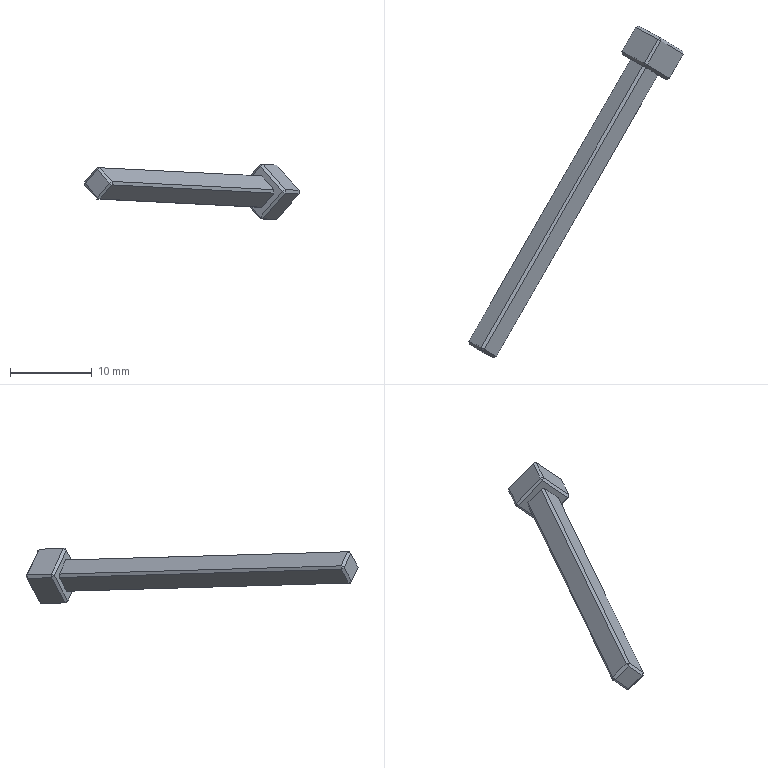Component | SolidWorks | 6z0-123-1 | 1 solid | 46 faces | box 26.14 x 40.54 x 6.74 mm | volume 422 mm3 | plane 44 | cylinder 2 | commonest cylinder face diameters 4.2 x2
STEP:
#1=COLOUR_RGB('',0.7922,0.8196,0.9333);
#2=FILL_AREA_STYLE_COLOUR('',#1);
#3=FILL_AREA_STYLE('',(#2));
#4=SURFACE_STYLE_FILL_AREA(#3);
#5=SURFACE_SIDE_STYLE('',(#4));
#6=SURFACE_STYLE_USAGE(.BOTH.,#5);
#7=PRESENTATION_STYLE_ASSIGNMENT((#6));
#8=CARTESIAN_POINT('',(-3.495,-3.817,3.283));
#9=VERTEX_POINT('',#8);
#10=CARTESIAN_POINT('',(-3.394,-3.878,3.168));
#11=VERTEX_POINT('',#10);
#12=CARTESIAN_POINT('',(-3.445,-3.847,3.225));
#13=DIRECTION('',(0.4977,0.867,-0.02519));
#14=DIRECTION('',(0.6119,-0.3716,-0.6982));
#15=AXIS2_PLACEMENT_3D('',#12,#13,#14);
#16=CIRCLE('',#15,0.08268);
#17=EDGE_CURVE('',#9,#11,#16,.T.);
#18=ORIENTED_EDGE('',*,*,#17,.F.);
#19=CARTESIAN_POINT('',(-3.456,-3.748,3.281));
#20=VERTEX_POINT('',#19);
#21=CARTESIAN_POINT('',(-3.495,-3.817,3.283));
#22=DIRECTION('',(0.4977,0.867,-0.02519));
#23=VECTOR('',#22,39.37);
#24=LINE('',#21,#23);
#25=EDGE_CURVE('',#9,#20,#24,.T.);
#26=ORIENTED_EDGE('',*,*,#25,.T.);
#27=CARTESIAN_POINT('',(-3.355,-3.81,3.166));
#28=VERTEX_POINT('',#27);
#29=CARTESIAN_POINT('',(-3.406,-3.779,3.223));
#30=DIRECTION('',(0.4977,0.867,-0.02519));
#31=DIRECTION('',(0.6119,-0.3716,-0.6982));
#32=AXIS2_PLACEMENT_3D('',#29,#30,#31);
#33=CIRCLE('',#32,0.08268);
#34=EDGE_CURVE('',#20,#28,#33,.T.);
#35=ORIENTED_EDGE('',*,*,#34,.T.);
#36=CARTESIAN_POINT('',(-3.394,-3.878,3.168));
#37=DIRECTION('',(0.4977,0.867,-0.02519));
#38=VECTOR('',#37,39.37);
#39=LINE('',#36,#38);
#40=EDGE_CURVE('',#11,#28,#39,.T.);
#41=ORIENTED_EDGE('',*,*,#40,.F.);
#42=EDGE_LOOP('',(#18,#26,#35,#41));
#43=FACE_OUTER_BOUND('',#42,.T.);
#44=CARTESIAN_POINT('',(-3.445,-3.847,3.225));
#45=DIRECTION('',(0.4977,0.867,-0.02519));
#46=DIRECTION('',(0.6119,-0.3716,-0.6982));
#47=AXIS2_PLACEMENT_3D('',#44,#45,#46);
#48=CYLINDRICAL_SURFACE('',#47,0.08268);
#49=ADVANCED_FACE('',(#43),#48,.F.);
#50=CARTESIAN_POINT('',(-3.484,-3.919,3.105));
#51=VERTEX_POINT('',#50);
#52=CARTESIAN_POINT('',(-3.378,-3.977,3.229));
#53=VERTEX_POINT('',#52);
#54=CARTESIAN_POINT('',(-3.371,-3.981,3.237));
#55=DIRECTION('',(0.6147,-0.3321,0.7154));
#56=VECTOR('',#55,39.37);
#57=LINE('',#54,#56);
#58=EDGE_CURVE('',#51,#53,#57,.T.);
#59=ORIENTED_EDGE('',*,*,#58,.T.);
#60=CARTESIAN_POINT('',(-3.484,-3.912,3.35));
#61=VERTEX_POINT('',#60);
#62=CARTESIAN_POINT('',(-3.491,-3.908,3.358));
#63=DIRECTION('',(-0.6119,0.3716,0.6982));
#64=VECTOR('',#63,39.37);
#65=LINE('',#62,#64);
#66=EDGE_CURVE('',#53,#61,#65,.T.);
#67=ORIENTED_EDGE('',*,*,#66,.T.);
#68=CARTESIAN_POINT('',(-3.59,-3.855,3.226));
#69=VERTEX_POINT('',#68);
#70=CARTESIAN_POINT('',(-3.598,-3.851,3.217));
#71=DIRECTION('',(-0.6147,0.3321,-0.7154));
#72=VECTOR('',#71,39.37);
#73=LINE('',#70,#72);
#74=EDGE_CURVE('',#61,#69,#73,.T.);
#75=ORIENTED_EDGE('',*,*,#74,.T.);
#76=CARTESIAN_POINT('',(-3.477,-3.924,3.097));
#77=DIRECTION('',(0.6119,-0.3716,-0.6982));
#78=VECTOR('',#77,39.37);
#79=LINE('',#76,#78);
#80=EDGE_CURVE('',#69,#51,#79,.T.);
#81=ORIENTED_EDGE('',*,*,#80,.T.);
#82=EDGE_LOOP('',(#59,#67,#75,#81));
#83=FACE_OUTER_BOUND('',#82,.T.);
#84=CARTESIAN_POINT('',(-3.549,-3.879,3.218));
#85=VERTEX_POINT('',#84);
#86=CARTESIAN_POINT('',(-3.491,-3.914,3.152));
#87=VERTEX_POINT('',#86);
#88=CARTESIAN_POINT('',(-3.484,-3.918,3.144));
#89=DIRECTION('',(0.6119,-0.3716,-0.6982));
#90=VECTOR('',#89,39.37);
#91=LINE('',#88,#90);
#92=EDGE_CURVE('',#85,#87,#91,.T.);
#93=ORIENTED_EDGE('',*,*,#92,.F.);
#94=CARTESIAN_POINT('',(-3.549,-3.878,3.235));
#95=VERTEX_POINT('',#94);
#96=CARTESIAN_POINT('',(-3.549,-3.879,3.218));
#97=DIRECTION('',(0.001966,0.02792,0.9996));
#98=VECTOR('',#97,39.37);
#99=LINE('',#96,#98);
#100=EDGE_CURVE('',#85,#95,#99,.T.);
#101=ORIENTED_EDGE('',*,*,#100,.T.);
#102=CARTESIAN_POINT('',(-3.491,-3.909,3.302));
#103=VERTEX_POINT('',#102);
#104=CARTESIAN_POINT('',(-3.556,-3.874,3.226));
#105=DIRECTION('',(-0.6147,0.3321,-0.7154));
#106=VECTOR('',#105,39.37);
#107=LINE('',#104,#106);
#108=EDGE_CURVE('',#103,#95,#107,.T.);
#109=ORIENTED_EDGE('',*,*,#108,.F.);
#110=CARTESIAN_POINT('',(-3.477,-3.918,3.302));
#111=VERTEX_POINT('',#110);
#112=CARTESIAN_POINT('',(-3.491,-3.909,3.302));
#113=DIRECTION('',(0.8673,-0.4976,0.01219));
#114=VECTOR('',#113,39.37);
#115=LINE('',#112,#114);
#116=EDGE_CURVE('',#103,#111,#115,.T.);
#117=ORIENTED_EDGE('',*,*,#116,.T.);
#118=CARTESIAN_POINT('',(-3.419,-3.953,3.237));
#119=VERTEX_POINT('',#118);
#120=CARTESIAN_POINT('',(-3.412,-3.957,3.228));
#121=DIRECTION('',(-0.6119,0.3716,0.6982));
#122=VECTOR('',#121,39.37);
#123=LINE('',#120,#122);
#124=EDGE_CURVE('',#119,#111,#123,.T.);
#125=ORIENTED_EDGE('',*,*,#124,.F.);
#126=CARTESIAN_POINT('',(-3.419,-3.953,3.22));
#127=VERTEX_POINT('',#126);
#128=CARTESIAN_POINT('',(-3.419,-3.953,3.237));
#129=DIRECTION('',(-0.001966,-0.02792,-0.9996));
#130=VECTOR('',#129,39.37);
#131=LINE('',#128,#130);
#132=EDGE_CURVE('',#119,#127,#131,.T.);
#133=ORIENTED_EDGE('',*,*,#132,.T.);
#134=CARTESIAN_POINT('',(-3.477,-3.922,3.152));
#135=VERTEX_POINT('',#134);
#136=CARTESIAN_POINT('',(-3.484,-3.918,3.144));
#137=DIRECTION('',(0.6147,-0.3321,0.7154));
#138=VECTOR('',#137,39.37);
#139=LINE('',#136,#138);
#140=EDGE_CURVE('',#135,#127,#139,.T.);
#141=ORIENTED_EDGE('',*,*,#140,.F.);
#142=CARTESIAN_POINT('',(-3.477,-3.922,3.152));
#143=DIRECTION('',(-0.8673,0.4976,-0.01219));
#144=VECTOR('',#143,39.37);
#145=LINE('',#142,#144);
#146=EDGE_CURVE('',#135,#87,#145,.T.);
#147=ORIENTED_EDGE('',*,*,#146,.T.);
#148=EDGE_LOOP('',(#93,#101,#109,#117,#125,#133,#141,#147));
#149=FACE_BOUND('',#148,.T.);
#150=CARTESIAN_POINT('',(-3.484,-3.916,3.227));
#151=DIRECTION('',(-0.4977,-0.867,0.02519));
#152=DIRECTION('',(-0.6119,0.3716,0.6982));
#153=AXIS2_PLACEMENT_3D('',#150,#151,#152);
#154=PLANE('',#153);
#155=ADVANCED_FACE('',(#83,#149),#154,.T.);
#156=CARTESIAN_POINT('',(-3.525,-3.724,3.23));
#157=VERTEX_POINT('',#156);
#158=CARTESIAN_POINT('',(-3.592,-3.84,3.234));
#159=VERTEX_POINT('',#158);
#160=CARTESIAN_POINT('',(-3.598,-3.85,3.234));
#161=DIRECTION('',(-0.4977,-0.867,0.02519));
#162=VECTOR('',#161,39.37);
#163=LINE('',#160,#162);
#164=EDGE_CURVE('',#157,#159,#163,.T.);
#165=ORIENTED_EDGE('',*,*,#164,.T.);
#166=CARTESIAN_POINT('',(-3.485,-3.898,3.358));
#167=VERTEX_POINT('',#166);
#168=CARTESIAN_POINT('',(-3.478,-3.902,3.366));
#169=DIRECTION('',(0.6147,-0.3321,0.7154));
#170=VECTOR('',#169,39.37);
#171=LINE('',#168,#170);
#172=EDGE_CURVE('',#159,#167,#171,.T.);
#173=ORIENTED_EDGE('',*,*,#172,.T.);
#174=CARTESIAN_POINT('',(-3.419,-3.782,3.354));
#175=VERTEX_POINT('',#174);
#176=CARTESIAN_POINT('',(-3.491,-3.908,3.358));
#177=DIRECTION('',(0.4977,0.867,-0.02519));
#178=VECTOR('',#177,39.37);
#179=LINE('',#176,#178);
#180=EDGE_CURVE('',#167,#175,#179,.T.);
#181=ORIENTED_EDGE('',*,*,#180,.T.);
#182=CARTESIAN_POINT('',(-3.532,-3.72,3.222));
#183=DIRECTION('',(-0.6147,0.3321,-0.7154));
#184=VECTOR('',#183,39.37);
#185=LINE('',#182,#184);
#186=EDGE_CURVE('',#175,#157,#185,.T.);
#187=ORIENTED_EDGE('',*,*,#186,.T.);
#188=EDGE_LOOP('',(#165,#173,#181,#187));
#189=FACE_OUTER_BOUND('',#188,.T.);
#190=CARTESIAN_POINT('',(-3.605,-3.846,3.226));
#191=DIRECTION('',(0.6119,-0.3716,-0.6982));
#192=DIRECTION('',(0.6147,-0.3321,0.7154));
#193=AXIS2_PLACEMENT_3D('',#190,#191,#192);
#194=PLANE('',#193);
#195=ADVANCED_FACE('',(#189),#194,.F.);
#196=CARTESIAN_POINT('',(-3.486,-3.905,3.096));
#197=VERTEX_POINT('',#196);
#198=CARTESIAN_POINT('',(-3.592,-3.841,3.217));
#199=VERTEX_POINT('',#198);
#200=CARTESIAN_POINT('',(-3.599,-3.836,3.225));
#201=DIRECTION('',(-0.6119,0.3716,0.6982));
#202=VECTOR('',#201,39.37);
#203=LINE('',#200,#202);
#204=EDGE_CURVE('',#197,#199,#203,.T.);
#205=ORIENTED_EDGE('',*,*,#204,.T.);
#206=CARTESIAN_POINT('',(-3.525,-3.725,3.214));
#207=VERTEX_POINT('',#206);
#208=CARTESIAN_POINT('',(-3.598,-3.851,3.217));
#209=DIRECTION('',(0.4977,0.867,-0.02519));
#210=VECTOR('',#209,39.37);
#211=LINE('',#208,#210);
#212=EDGE_CURVE('',#199,#207,#211,.T.);
#213=ORIENTED_EDGE('',*,*,#212,.T.);
#214=CARTESIAN_POINT('',(-3.419,-3.789,3.093));
#215=VERTEX_POINT('',#214);
#216=CARTESIAN_POINT('',(-3.412,-3.793,3.084));
#217=DIRECTION('',(0.6119,-0.3716,-0.6982));
#218=VECTOR('',#217,39.37);
#219=LINE('',#216,#218);
#220=EDGE_CURVE('',#207,#215,#219,.T.);
#221=ORIENTED_EDGE('',*,*,#220,.T.);
#222=CARTESIAN_POINT('',(-3.492,-3.915,3.096));
#223=DIRECTION('',(-0.4977,-0.867,0.02519));
#224=VECTOR('',#223,39.37);
#225=LINE('',#222,#224);
#226=EDGE_CURVE('',#215,#197,#225,.T.);
#227=ORIENTED_EDGE('',*,*,#226,.T.);
#228=EDGE_LOOP('',(#205,#213,#221,#227));
#229=FACE_OUTER_BOUND('',#228,.T.);
#230=CARTESIAN_POINT('',(-3.484,-3.92,3.088));
#231=DIRECTION('',(0.6147,-0.3321,0.7154));
#232=DIRECTION('',(0.4977,0.867,-0.02519));
#233=AXIS2_PLACEMENT_3D('',#230,#231,#232);
#234=PLANE('',#233);
#235=ADVANCED_FACE('',(#229),#234,.F.);
#236=CARTESIAN_POINT('',(-3.405,-3.797,3.093));
#237=VERTEX_POINT('',#236);
#238=CARTESIAN_POINT('',(-3.298,-3.855,3.217));
#239=VERTEX_POINT('',#238);
#240=CARTESIAN_POINT('',(-3.412,-3.793,3.084));
#241=DIRECTION('',(0.6147,-0.3321,0.7154));
#242=VECTOR('',#241,39.37);
#243=LINE('',#240,#242);
#244=EDGE_CURVE('',#237,#239,#243,.T.);
#245=ORIENTED_EDGE('',*,*,#244,.T.);
#246=CARTESIAN_POINT('',(-3.365,-3.971,3.22));
#247=VERTEX_POINT('',#246);
#248=CARTESIAN_POINT('',(-3.371,-3.981,3.22));
#249=DIRECTION('',(-0.4977,-0.867,0.02519));
#250=VECTOR('',#249,39.37);
#251=LINE('',#248,#250);
#252=EDGE_CURVE('',#239,#247,#251,.T.);
#253=ORIENTED_EDGE('',*,*,#252,.T.);
#254=CARTESIAN_POINT('',(-3.471,-3.913,3.096));
#255=VERTEX_POINT('',#254);
#256=CARTESIAN_POINT('',(-3.478,-3.909,3.088));
#257=DIRECTION('',(-0.6147,0.3321,-0.7154));
#258=VECTOR('',#257,39.37);
#259=LINE('',#256,#258);
#260=EDGE_CURVE('',#247,#255,#259,.T.);
#261=ORIENTED_EDGE('',*,*,#260,.T.);
#262=CARTESIAN_POINT('',(-3.477,-3.924,3.097));
#263=DIRECTION('',(0.4977,0.867,-0.02519));
#264=VECTOR('',#263,39.37);
#265=LINE('',#262,#264);
#266=EDGE_CURVE('',#255,#237,#265,.T.);
#267=ORIENTED_EDGE('',*,*,#266,.T.);
#268=EDGE_LOOP('',(#245,#253,#261,#267));
#269=FACE_OUTER_BOUND('',#268,.T.);
#270=CARTESIAN_POINT('',(-3.484,-3.92,3.088));
#271=DIRECTION('',(-0.6119,0.3716,0.6982));
#272=DIRECTION('',(-0.6147,0.3321,-0.7154));
#273=AXIS2_PLACEMENT_3D('',#270,#271,#272);
#274=PLANE('',#273);
#275=ADVANCED_FACE('',(#269),#274,.F.);
#276=CARTESIAN_POINT('',(-3.471,-3.906,3.358));
#277=VERTEX_POINT('',#276);
#278=CARTESIAN_POINT('',(-3.365,-3.97,3.237));
#279=VERTEX_POINT('',#278);
#280=CARTESIAN_POINT('',(-3.357,-3.975,3.229));
#281=DIRECTION('',(0.6119,-0.3716,-0.6982));
#282=VECTOR('',#281,39.37);
#283=LINE('',#280,#282);
#284=EDGE_CURVE('',#277,#279,#283,.T.);
#285=ORIENTED_EDGE('',*,*,#284,.T.);
#286=CARTESIAN_POINT('',(-3.298,-3.854,3.234));
#287=VERTEX_POINT('',#286);
#288=CARTESIAN_POINT('',(-3.371,-3.981,3.237));
#289=DIRECTION('',(0.4977,0.867,-0.02519));
#290=VECTOR('',#289,39.37);
#291=LINE('',#288,#290);
#292=EDGE_CURVE('',#279,#287,#291,.T.);
#293=ORIENTED_EDGE('',*,*,#292,.T.);
#294=CARTESIAN_POINT('',(-3.404,-3.79,3.354));
#295=VERTEX_POINT('',#294);
#296=CARTESIAN_POINT('',(-3.291,-3.859,3.225));
#297=DIRECTION('',(-0.6119,0.3716,0.6982));
#298=VECTOR('',#297,39.37);
#299=LINE('',#296,#298);
#300=EDGE_CURVE('',#287,#295,#299,.T.);
#301=ORIENTED_EDGE('',*,*,#300,.T.);
#302=CARTESIAN_POINT('',(-3.477,-3.916,3.358));
#303=DIRECTION('',(-0.4977,-0.867,0.02519));
#304=VECTOR('',#303,39.37);
#305=LINE('',#302,#304);
#306=EDGE_CURVE('',#295,#277,#305,.T.);
#307=ORIENTED_EDGE('',*,*,#306,.T.);
#308=EDGE_LOOP('',(#285,#293,#301,#307));
#309=FACE_OUTER_BOUND('',#308,.T.);
#310=CARTESIAN_POINT('',(-3.363,-3.985,3.229));
#311=DIRECTION('',(-0.6147,0.3321,-0.7154));
#312=DIRECTION('',(-0.4977,-0.867,0.02519));
#313=AXIS2_PLACEMENT_3D('',#310,#311,#312);
#314=PLANE('',#313);
#315=ADVANCED_FACE('',(#309),#314,.F.);
#316=CARTESIAN_POINT('',(-3.512,-3.718,3.222));
#317=VERTEX_POINT('',#316);
#318=CARTESIAN_POINT('',(-3.405,-3.776,3.346));
#319=VERTEX_POINT('',#318);
#320=CARTESIAN_POINT('',(-3.459,-3.747,3.284));
#321=DIRECTION('',(0.6147,-0.3321,0.7154));
#322=VECTOR('',#321,39.37);
#323=LINE('',#320,#322);
#324=EDGE_CURVE('',#317,#319,#323,.T.);
#325=ORIENTED_EDGE('',*,*,#324,.T.);
#326=CARTESIAN_POINT('',(-3.299,-3.84,3.225));
#327=VERTEX_POINT('',#326);
#328=CARTESIAN_POINT('',(-3.352,-3.808,3.285));
#329=DIRECTION('',(0.6119,-0.3716,-0.6982));
#330=VECTOR('',#329,39.37);
#331=LINE('',#328,#330);
#332=EDGE_CURVE('',#319,#327,#331,.T.);
#333=ORIENTED_EDGE('',*,*,#332,.T.);
#334=CARTESIAN_POINT('',(-3.406,-3.783,3.101));
#335=VERTEX_POINT('',#334);
#336=CARTESIAN_POINT('',(-3.353,-3.811,3.163));
#337=DIRECTION('',(-0.6147,0.3321,-0.7154));
#338=VECTOR('',#337,39.37);
#339=LINE('',#336,#338);
#340=EDGE_CURVE('',#327,#335,#339,.T.);
#341=ORIENTED_EDGE('',*,*,#340,.T.);
#342=CARTESIAN_POINT('',(-3.459,-3.75,3.161));
#343=DIRECTION('',(-0.6119,0.3716,0.6982));
#344=VECTOR('',#343,39.37);
#345=LINE('',#342,#344);
#346=EDGE_CURVE('',#335,#317,#345,.T.);
#347=ORIENTED_EDGE('',*,*,#346,.T.);
#348=EDGE_LOOP('',(#325,#333,#341,#347));
#349=FACE_OUTER_BOUND('',#348,.T.);
#350=CARTESIAN_POINT('',(-3.406,-3.779,3.223));
#351=DIRECTION('',(0.4977,0.867,-0.02519));
#352=DIRECTION('',(0.6119,-0.3716,-0.6982));
#353=AXIS2_PLACEMENT_3D('',#350,#351,#352);
#354=CIRCLE('',#353,0.08268);
#355=EDGE_CURVE('',#28,#20,#354,.T.);
#356=ORIENTED_EDGE('',*,*,#355,.F.);
#357=ORIENTED_EDGE('',*,*,#34,.F.);
#358=EDGE_LOOP('',(#356,#357));
#359=FACE_BOUND('',#358,.T.);
#360=CARTESIAN_POINT('',(-3.406,-3.779,3.223));
#361=DIRECTION('',(-0.4977,-0.867,0.02519));
#362=DIRECTION('',(-0.6119,0.3716,0.6982));
#363=AXIS2_PLACEMENT_3D('',#360,#361,#362);
#364=PLANE('',#363);
#365=ADVANCED_FACE('',(#349,#359),#364,.F.);
#366=CARTESIAN_POINT('',(-4.327,-5.233,3.274));
#367=VERTEX_POINT('',#366);
#368=CARTESIAN_POINT('',(-4.269,-5.265,3.342));
#369=VERTEX_POINT('',#368);
#370=CARTESIAN_POINT('',(-4.262,-5.268,3.35));
#371=DIRECTION('',(0.6147,-0.3321,0.7154));
#372=VECTOR('',#371,39.37);
#373=LINE('',#370,#372);
#374=EDGE_CURVE('',#367,#369,#373,.T.);
#375=ORIENTED_EDGE('',*,*,#374,.T.);
#376=CARTESIAN_POINT('',(-4.275,-5.275,3.342));
#377=DIRECTION('',(0.4977,0.867,-0.02519));
#378=VECTOR('',#377,39.37);
#379=LINE('',#376,#378);
#380=EDGE_CURVE('',#369,#103,#379,.T.);
#381=ORIENTED_EDGE('',*,*,#380,.T.);
#382=ORIENTED_EDGE('',*,*,#108,.T.);
#383=CARTESIAN_POINT('',(-4.333,-5.243,3.274));
#384=DIRECTION('',(-0.4977,-0.867,0.02519));
#385=VECTOR('',#384,39.37);
#386=LINE('',#383,#385);
#387=EDGE_CURVE('',#95,#367,#386,.T.);
#388=ORIENTED_EDGE('',*,*,#387,.T.);
#389=EDGE_LOOP('',(#375,#381,#382,#388));
#390=FACE_OUTER_BOUND('',#389,.T.);
#391=CARTESIAN_POINT('',(-4.34,-5.239,3.266));
#392=DIRECTION('',(0.6119,-0.3716,-0.6982));
#393=DIRECTION('',(0.6147,-0.3321,0.7154));
#394=AXIS2_PLACEMENT_3D('',#391,#392,#393);
#395=PLANE('',#394);
#396=ADVANCED_FACE('',(#390),#395,.F.);
#397=ORIENTED_EDGE('',*,*,#92,.T.);
#398=CARTESIAN_POINT('',(-4.269,-5.269,3.191));
#399=VERTEX_POINT('',#398);
#400=CARTESIAN_POINT('',(-4.275,-5.279,3.192));
#401=DIRECTION('',(-0.4977,-0.867,0.02519));
#402=VECTOR('',#401,39.37);
#403=LINE('',#400,#402);
#404=EDGE_CURVE('',#87,#399,#403,.T.);
#405=ORIENTED_EDGE('',*,*,#404,.T.);
#406=CARTESIAN_POINT('',(-4.327,-5.234,3.257));
#407=VERTEX_POINT('',#406);
#408=CARTESIAN_POINT('',(-4.334,-5.229,3.266));
#409=DIRECTION('',(-0.6119,0.3716,0.6982));
#410=VECTOR('',#409,39.37);
#411=LINE('',#408,#410);
#412=EDGE_CURVE('',#399,#407,#411,.T.);
#413=ORIENTED_EDGE('',*,*,#412,.T.);
#414=CARTESIAN_POINT('',(-4.333,-5.244,3.258));
#415=DIRECTION('',(0.4977,0.867,-0.02519));
#416=VECTOR('',#415,39.37);
#417=LINE('',#414,#416);
#418=EDGE_CURVE('',#407,#85,#417,.T.);
#419=ORIENTED_EDGE('',*,*,#418,.T.);
#420=EDGE_LOOP('',(#397,#405,#413,#419));
#421=FACE_OUTER_BOUND('',#420,.T.);
#422=CARTESIAN_POINT('',(-4.268,-5.283,3.183));
#423=DIRECTION('',(0.6147,-0.3321,0.7154));
#424=DIRECTION('',(0.4977,0.867,-0.02519));
#425=AXIS2_PLACEMENT_3D('',#422,#423,#424);
#426=PLANE('',#425);
#427=ADVANCED_FACE('',(#421),#426,.F.);
#428=ORIENTED_EDGE('',*,*,#140,.T.);
#429=CARTESIAN_POINT('',(-4.197,-5.308,3.259));
#430=VERTEX_POINT('',#429);
#431=CARTESIAN_POINT('',(-4.203,-5.319,3.259));
#432=DIRECTION('',(-0.4977,-0.867,0.02519));
#433=VECTOR('',#432,39.37);
#434=LINE('',#431,#433);
#435=EDGE_CURVE('',#127,#430,#434,.T.);
#436=ORIENTED_EDGE('',*,*,#435,.T.);
#437=CARTESIAN_POINT('',(-4.255,-5.277,3.192));
#438=VERTEX_POINT('',#437);
#439=CARTESIAN_POINT('',(-4.262,-5.273,3.183));
#440=DIRECTION('',(-0.6147,0.3321,-0.7154));
#441=VECTOR('',#440,39.37);
#442=LINE('',#439,#441);
#443=EDGE_CURVE('',#430,#438,#442,.T.);
#444=ORIENTED_EDGE('',*,*,#443,.T.);
#445=CARTESIAN_POINT('',(-4.261,-5.287,3.192));
#446=DIRECTION('',(0.4977,0.867,-0.02519));
#447=VECTOR('',#446,39.37);
#448=LINE('',#445,#447);
#449=EDGE_CURVE('',#438,#135,#448,.T.);
#450=ORIENTED_EDGE('',*,*,#449,.T.);
#451=EDGE_LOOP('',(#428,#436,#444,#450));
#452=FACE_OUTER_BOUND('',#451,.T.);
#453=CARTESIAN_POINT('',(-4.268,-5.283,3.183));
#454=DIRECTION('',(-0.6119,0.3716,0.6982));
#455=DIRECTION('',(-0.6147,0.3321,-0.7154));
#456=AXIS2_PLACEMENT_3D('',#453,#454,#455);
#457=PLANE('',#456);
#458=ADVANCED_FACE('',(#452),#457,.F.);
#459=CARTESIAN_POINT('',(-4.255,-5.273,3.342));
#460=VERTEX_POINT('',#459);
#461=CARTESIAN_POINT('',(-4.197,-5.308,3.276));
#462=VERTEX_POINT('',#461);
#463=CARTESIAN_POINT('',(-4.19,-5.312,3.268));
#464=DIRECTION('',(0.6119,-0.3716,-0.6982));
#465=VECTOR('',#464,39.37);
#466=LINE('',#463,#465);
#467=EDGE_CURVE('',#460,#462,#466,.T.);
#468=ORIENTED_EDGE('',*,*,#467,.T.);
#469=CARTESIAN_POINT('',(-4.203,-5.318,3.276));
#470=DIRECTION('',(0.4977,0.867,-0.02519));
#471=VECTOR('',#470,39.37);
#472=LINE('',#469,#471);
#473=EDGE_CURVE('',#462,#119,#472,.T.);
#474=ORIENTED_EDGE('',*,*,#473,.T.);
#475=ORIENTED_EDGE('',*,*,#124,.T.);
#476=CARTESIAN_POINT('',(-4.26,-5.283,3.342));
#477=DIRECTION('',(-0.4977,-0.867,0.02519));
#478=VECTOR('',#477,39.37);
#479=LINE('',#476,#478);
#480=EDGE_CURVE('',#111,#460,#479,.T.);
#481=ORIENTED_EDGE('',*,*,#480,.T.);
#482=EDGE_LOOP('',(#468,#474,#475,#481));
#483=FACE_OUTER_BOUND('',#482,.T.);
#484=CARTESIAN_POINT('',(-4.195,-5.323,3.268));
#485=DIRECTION('',(-0.6147,0.3321,-0.7154));
#486=DIRECTION('',(-0.4977,-0.867,0.02519));
#487=AXIS2_PLACEMENT_3D('',#484,#485,#486);
#488=PLANE('',#487);
#489=ADVANCED_FACE('',(#483),#488,.F.);
#490=CARTESIAN_POINT('',(-4.268,-5.279,3.334));
#491=VERTEX_POINT('',#490);
#492=CARTESIAN_POINT('',(-4.326,-5.248,3.266));
#493=VERTEX_POINT('',#492);
#494=CARTESIAN_POINT('',(-4.333,-5.244,3.258));
#495=DIRECTION('',(-0.6147,0.3321,-0.7154));
#496=VECTOR('',#495,39.37);
#497=LINE('',#494,#496);
#498=EDGE_CURVE('',#491,#493,#497,.T.);
#499=ORIENTED_EDGE('',*,*,#498,.T.);
#500=CARTESIAN_POINT('',(-4.268,-5.283,3.2));
#501=VERTEX_POINT('',#500);
#502=CARTESIAN_POINT('',(-4.261,-5.287,3.192));
#503=DIRECTION('',(0.6119,-0.3716,-0.6982));
#504=VECTOR('',#503,39.37);
#505=LINE('',#502,#504);
#506=EDGE_CURVE('',#493,#501,#505,.T.);
#507=ORIENTED_EDGE('',*,*,#506,.T.);
#508=CARTESIAN_POINT('',(-4.21,-5.314,3.268));
#509=VERTEX_POINT('',#508);
#510=CARTESIAN_POINT('',(-4.203,-5.318,3.276));
#511=DIRECTION('',(0.6147,-0.3321,0.7154));
#512=VECTOR('',#511,39.37);
#513=LINE('',#510,#512);
#514=EDGE_CURVE('',#501,#509,#513,.T.);
#515=ORIENTED_EDGE('',*,*,#514,.T.);
#516=CARTESIAN_POINT('',(-4.275,-5.275,3.342));
#517=DIRECTION('',(-0.6119,0.3716,0.6982));
#518=VECTOR('',#517,39.37);
#519=LINE('',#516,#518);
#520=EDGE_CURVE('',#509,#491,#519,.T.);
#521=ORIENTED_EDGE('',*,*,#520,.T.);
#522=EDGE_LOOP('',(#499,#507,#515,#521));
#523=FACE_OUTER_BOUND('',#522,.T.);
#524=CARTESIAN_POINT('',(-4.268,-5.281,3.267));
#525=DIRECTION('',(-0.4977,-0.867,0.02519));
#526=DIRECTION('',(-0.6119,0.3716,0.6982));
#527=AXIS2_PLACEMENT_3D('',#524,#525,#526);
#528=PLANE('',#527);
#529=ADVANCED_FACE('',(#523),#528,.T.);
#530=ORIENTED_EDGE('',*,*,#25,.F.);
#531=CARTESIAN_POINT('',(-3.445,-3.847,3.225));
#532=DIRECTION('',(0.4977,0.867,-0.02519));
#533=DIRECTION('',(0.6119,-0.3716,-0.6982));
#534=AXIS2_PLACEMENT_3D('',#531,#532,#533);
#535=CIRCLE('',#534,0.08268);
#536=EDGE_CURVE('',#11,#9,#535,.T.);
#537=ORIENTED_EDGE('',*,*,#536,.F.);
#538=ORIENTED_EDGE('',*,*,#40,.T.);
#539=ORIENTED_EDGE('',*,*,#355,.T.);
#540=EDGE_LOOP('',(#530,#537,#538,#539));
#541=FACE_OUTER_BOUND('',#540,.T.);
#542=CARTESIAN_POINT('',(-3.445,-3.847,3.225));
#543=DIRECTION('',(0.4977,0.867,-0.02519));
#544=DIRECTION('',(0.6119,-0.3716,-0.6982));
#545=AXIS2_PLACEMENT_3D('',#542,#543,#544);
#546=CYLINDRICAL_SURFACE('',#545,0.08268);
#547=ADVANCED_FACE('',(#541),#546,.F.);
#548=ORIENTED_EDGE('',*,*,#536,.T.);
#549=ORIENTED_EDGE('',*,*,#17,.T.);
#550=EDGE_LOOP('',(#548,#549));
#551=FACE_OUTER_BOUND('',#550,.T.);
#552=CARTESIAN_POINT('',(-3.445,-3.847,3.225));
#553=DIRECTION('',(0.4977,0.867,-0.02519));
#554=DIRECTION('',(0.6119,-0.3716,-0.6982));
#555=AXIS2_PLACEMENT_3D('',#552,#553,#554);
#556=PLANE('',#555);
#557=ADVANCED_FACE('',(#551),#556,.T.);
#558=ORIENTED_EDGE('',*,*,#116,.F.);
#559=ORIENTED_EDGE('',*,*,#380,.F.);
#560=CARTESIAN_POINT('',(-4.262,-5.269,3.342));
#561=DIRECTION('',(-0.8673,0.4976,-0.01219));
#562=VECTOR('',#561,39.37);
#563=LINE('',#560,#562);
#564=EDGE_CURVE('',#460,#369,#563,.T.);
#565=ORIENTED_EDGE('',*,*,#564,.F.);
#566=ORIENTED_EDGE('',*,*,#480,.F.);
#567=EDGE_LOOP('',(#558,#559,#565,#566));
#568=FACE_OUTER_BOUND('',#567,.T.);
#569=CARTESIAN_POINT('',(-4.275,-5.275,3.342));
#570=DIRECTION('',(-0.001966,-0.02792,-0.9996));
#571=DIRECTION('',(0.4977,0.867,-0.02519));
#572=AXIS2_PLACEMENT_3D('',#569,#570,#571);
#573=PLANE('',#572);
#574=ADVANCED_FACE('',(#568),#573,.F.);
#575=CARTESIAN_POINT('',(-4.203,-5.311,3.272));
#576=DIRECTION('',(-0.7866,-0.3782,-0.4881));
#577=VECTOR('',#576,39.37);
#578=LINE('',#575,#577);
#579=EDGE_CURVE('',#462,#509,#578,.T.);
#580=ORIENTED_EDGE('',*,*,#579,.F.);
#581=ORIENTED_EDGE('',*,*,#467,.F.);
#582=CARTESIAN_POINT('',(-4.268,-5.279,3.334));
#583=DIRECTION('',(0.7866,0.3782,0.4881));
#584=VECTOR('',#583,39.37);
#585=LINE('',#582,#584);
#586=EDGE_CURVE('',#491,#460,#585,.T.);
#587=ORIENTED_EDGE('',*,*,#586,.F.);
#588=ORIENTED_EDGE('',*,*,#520,.F.);
#589=EDGE_LOOP('',(#580,#581,#587,#588));
#590=FACE_OUTER_BOUND('',#589,.T.);
#591=CARTESIAN_POINT('',(-4.239,-5.297,3.301));
#592=DIRECTION('',(0.08272,-0.8479,0.5237));
#593=DIRECTION('',(0.6119,-0.3716,-0.6982));
#594=AXIS2_PLACEMENT_3D('',#591,#592,#593);
#595=PLANE('',#594);
#596=ADVANCED_FACE('',(#590),#595,.T.);
#597=ORIENTED_EDGE('',*,*,#132,.F.);
#598=ORIENTED_EDGE('',*,*,#473,.F.);
#599=CARTESIAN_POINT('',(-4.197,-5.308,3.259));
#600=DIRECTION('',(0.001966,0.02792,0.9996));
#601=VECTOR('',#600,39.37);
#602=LINE('',#599,#601);
#603=EDGE_CURVE('',#430,#462,#602,.T.);
#604=ORIENTED_EDGE('',*,*,#603,.F.);
#605=ORIENTED_EDGE('',*,*,#435,.F.);
#606=EDGE_LOOP('',(#597,#598,#604,#605));
#607=FACE_OUTER_BOUND('',#606,.T.);
#608=CARTESIAN_POINT('',(-4.203,-5.318,3.276));
#609=DIRECTION('',(-0.8673,0.4976,-0.01219));
#610=DIRECTION('',(0.4977,0.867,-0.02519));
#611=AXIS2_PLACEMENT_3D('',#608,#609,#610);
#612=PLANE('',#611);
#613=ADVANCED_FACE('',(#607),#612,.F.);
#614=ORIENTED_EDGE('',*,*,#586,.T.);
#615=ORIENTED_EDGE('',*,*,#564,.T.);
#616=CARTESIAN_POINT('',(-4.268,-5.279,3.334));
#617=DIRECTION('',(-0.08075,0.8758,0.4759));
#618=VECTOR('',#617,39.37);
#619=LINE('',#616,#618);
#620=EDGE_CURVE('',#491,#369,#619,.T.);
#621=ORIENTED_EDGE('',*,*,#620,.F.);
#622=EDGE_LOOP('',(#614,#615,#621));
#623=FACE_OUTER_BOUND('',#622,.T.);
#624=CARTESIAN_POINT('',(-4.268,-5.279,3.334));
#625=DIRECTION('',(-0.2857,-0.4778,0.8307));
#626=DIRECTION('',(-0.08075,0.8758,0.4759));
#627=AXIS2_PLACEMENT_3D('',#624,#625,#626);
#628=PLANE('',#627);
#629=ADVANCED_FACE('',(#623),#628,.T.);
#630=ORIENTED_EDGE('',*,*,#603,.T.);
#631=ORIENTED_EDGE('',*,*,#579,.T.);
#632=CARTESIAN_POINT('',(-4.197,-5.308,3.259));
#633=DIRECTION('',(-0.7846,-0.3503,0.5115));
#634=VECTOR('',#633,39.37);
#635=LINE('',#632,#634);
#636=EDGE_CURVE('',#430,#509,#635,.T.);
#637=ORIENTED_EDGE('',*,*,#636,.F.);
#638=EDGE_LOOP('',(#630,#631,#637));
#639=FACE_OUTER_BOUND('',#638,.T.);
#640=CARTESIAN_POINT('',(-4.197,-5.308,3.259));
#641=DIRECTION('',(0.4208,-0.9068,0.0245));
#642=DIRECTION('',(-0.7846,-0.3503,0.5115));
#643=AXIS2_PLACEMENT_3D('',#640,#641,#642);
#644=PLANE('',#643);
#645=ADVANCED_FACE('',(#639),#644,.T.);
#646=ORIENTED_EDGE('',*,*,#100,.F.);
#647=ORIENTED_EDGE('',*,*,#418,.F.);
#648=CARTESIAN_POINT('',(-4.327,-5.234,3.257));
#649=DIRECTION('',(-0.001966,-0.02792,-0.9996));
#650=VECTOR('',#649,39.37);
#651=LINE('',#648,#650);
#652=EDGE_CURVE('',#367,#407,#651,.T.);
#653=ORIENTED_EDGE('',*,*,#652,.F.);
#654=ORIENTED_EDGE('',*,*,#387,.F.);
#655=EDGE_LOOP('',(#646,#647,#653,#654));
#656=FACE_OUTER_BOUND('',#655,.T.);
#657=CARTESIAN_POINT('',(-4.333,-5.244,3.258));
#658=DIRECTION('',(0.8673,-0.4976,0.01219));
#659=DIRECTION('',(0.4977,0.867,-0.02519));
#660=AXIS2_PLACEMENT_3D('',#657,#658,#659);
#661=PLANE('',#660);
#662=ADVANCED_FACE('',(#656),#661,.F.);
#663=ORIENTED_EDGE('',*,*,#620,.T.);
#664=ORIENTED_EDGE('',*,*,#374,.F.);
#665=CARTESIAN_POINT('',(-4.326,-5.24,3.27));
#666=DIRECTION('',(-0.08075,0.8758,0.4759));
#667=VECTOR('',#666,39.37);
#668=LINE('',#665,#667);
#669=EDGE_CURVE('',#493,#367,#668,.T.);
#670=ORIENTED_EDGE('',*,*,#669,.F.);
#671=ORIENTED_EDGE('',*,*,#498,.F.);
#672=EDGE_LOOP('',(#663,#664,#670,#671));
#673=FACE_OUTER_BOUND('',#672,.T.);
#674=CARTESIAN_POINT('',(-4.297,-5.263,3.3));
#675=DIRECTION('',(-0.7846,-0.3503,0.5115));
#676=DIRECTION('',(0.6147,-0.3321,0.7154));
#677=AXIS2_PLACEMENT_3D('',#674,#675,#676);
#678=PLANE('',#677);
#679=ADVANCED_FACE('',(#673),#678,.T.);
#680=ORIENTED_EDGE('',*,*,#636,.T.);
#681=ORIENTED_EDGE('',*,*,#514,.F.);
#682=CARTESIAN_POINT('',(-4.268,-5.283,3.2));
#683=DIRECTION('',(-0.7846,-0.3503,0.5115));
#684=VECTOR('',#683,39.37);
#685=LINE('',#682,#684);
#686=EDGE_CURVE('',#438,#501,#685,.T.);
#687=ORIENTED_EDGE('',*,*,#686,.F.);
#688=ORIENTED_EDGE('',*,*,#443,.F.);
#689=EDGE_LOOP('',(#680,#681,#687,#688));
#690=FACE_OUTER_BOUND('',#689,.T.);
#691=CARTESIAN_POINT('',(-4.239,-5.299,3.234));
#692=DIRECTION('',(0.08075,-0.8758,-0.4759));
#693=DIRECTION('',(-0.6147,0.3321,-0.7154));
#694=AXIS2_PLACEMENT_3D('',#691,#692,#693);
#695=PLANE('',#694);
#696=ADVANCED_FACE('',(#690),#695,.T.);
#697=ORIENTED_EDGE('',*,*,#146,.F.);
#698=ORIENTED_EDGE('',*,*,#449,.F.);
#699=CARTESIAN_POINT('',(-4.262,-5.273,3.191));
#700=DIRECTION('',(0.8673,-0.4976,0.01219));
#701=VECTOR('',#700,39.37);
#702=LINE('',#699,#701);
#703=EDGE_CURVE('',#399,#438,#702,.T.);
#704=ORIENTED_EDGE('',*,*,#703,.F.);
#705=ORIENTED_EDGE('',*,*,#404,.F.);
#706=EDGE_LOOP('',(#697,#698,#704,#705));
#707=FACE_OUTER_BOUND('',#706,.T.);
#708=CARTESIAN_POINT('',(-4.261,-5.287,3.192));
#709=DIRECTION('',(0.001966,0.02792,0.9996));
#710=DIRECTION('',(0.4977,0.867,-0.02519));
#711=AXIS2_PLACEMENT_3D('',#708,#709,#710);
#712=PLANE('',#711);
#713=ADVANCED_FACE('',(#707),#712,.F.);
#714=ORIENTED_EDGE('',*,*,#669,.T.);
#715=ORIENTED_EDGE('',*,*,#652,.T.);
#716=CARTESIAN_POINT('',(-4.327,-5.234,3.257));
#717=DIRECTION('',(-0.08272,0.8479,-0.5237));
#718=VECTOR('',#717,39.37);
#719=LINE('',#716,#718);
#720=EDGE_CURVE('',#493,#407,#719,.T.);
#721=ORIENTED_EDGE('',*,*,#720,.F.);
#722=EDGE_LOOP('',(#714,#715,#721));
#723=FACE_OUTER_BOUND('',#722,.T.);
#724=CARTESIAN_POINT('',(-4.327,-5.234,3.257));
#725=DIRECTION('',(-0.9955,-0.09429,0.004591));
#726=DIRECTION('',(-0.08075,0.8758,0.4759));
#727=AXIS2_PLACEMENT_3D('',#724,#725,#726);
#728=PLANE('',#727);
#729=ADVANCED_FACE('',(#723),#728,.T.);
#730=ORIENTED_EDGE('',*,*,#703,.T.);
#731=ORIENTED_EDGE('',*,*,#686,.T.);
#732=CARTESIAN_POINT('',(-4.268,-5.283,3.2));
#733=DIRECTION('',(0.08272,-0.8479,0.5237));
#734=VECTOR('',#733,39.37);
#735=LINE('',#732,#734);
#736=EDGE_CURVE('',#399,#501,#735,.T.);
#737=ORIENTED_EDGE('',*,*,#736,.F.);
#738=EDGE_LOOP('',(#730,#731,#737));
#739=FACE_OUTER_BOUND('',#738,.T.);
#740=CARTESIAN_POINT('',(-4.268,-5.283,3.2));
#741=DIRECTION('',(-0.289,-0.5233,-0.8016));
#742=DIRECTION('',(-0.7846,-0.3503,0.5115));
#743=AXIS2_PLACEMENT_3D('',#740,#741,#742);
#744=PLANE('',#743);
#745=ADVANCED_FACE('',(#739),#744,.T.);
#746=ORIENTED_EDGE('',*,*,#720,.T.);
#747=ORIENTED_EDGE('',*,*,#412,.F.);
#748=ORIENTED_EDGE('',*,*,#736,.T.);
#749=ORIENTED_EDGE('',*,*,#506,.F.);
#750=EDGE_LOOP('',(#746,#747,#748,#749));
#751=FACE_OUTER_BOUND('',#750,.T.);
#752=CARTESIAN_POINT('',(-4.297,-5.265,3.233));
#753=DIRECTION('',(-0.7866,-0.3782,-0.4881));
#754=DIRECTION('',(-0.6119,0.3716,0.6982));
#755=AXIS2_PLACEMENT_3D('',#752,#753,#754);
#756=PLANE('',#755);
#757=ADVANCED_FACE('',(#751),#756,.T.);
#758=CARTESIAN_POINT('',(-3.592,-3.84,3.234));
#759=DIRECTION('',(-0.001966,-0.02792,-0.9996));
#760=VECTOR('',#759,39.37);
#761=LINE('',#758,#760);
#762=EDGE_CURVE('',#159,#199,#761,.T.);
#763=ORIENTED_EDGE('',*,*,#762,.F.);
#764=ORIENTED_EDGE('',*,*,#164,.F.);
#765=CARTESIAN_POINT('',(-3.525,-3.725,3.214));
#766=DIRECTION('',(0.001966,0.02792,0.9996));
#767=VECTOR('',#766,39.37);
#768=LINE('',#765,#767);
#769=EDGE_CURVE('',#207,#157,#768,.T.);
#770=ORIENTED_EDGE('',*,*,#769,.F.);
#771=ORIENTED_EDGE('',*,*,#212,.F.);
#772=EDGE_LOOP('',(#763,#764,#770,#771));
#773=FACE_OUTER_BOUND('',#772,.T.);
#774=CARTESIAN_POINT('',(-3.598,-3.851,3.217));
#775=DIRECTION('',(0.8673,-0.4976,0.01219));
#776=DIRECTION('',(0.4977,0.867,-0.02519));
#777=AXIS2_PLACEMENT_3D('',#774,#775,#776);
#778=PLANE('',#777);
#779=ADVANCED_FACE('',(#773),#778,.F.);
#780=CARTESIAN_POINT('',(-3.592,-3.84,3.234));
#781=DIRECTION('',(0.08075,-0.8758,-0.4759));
#782=VECTOR('',#781,39.37);
#783=LINE('',#780,#782);
#784=EDGE_CURVE('',#159,#69,#783,.T.);
#785=ORIENTED_EDGE('',*,*,#784,.F.);
#786=ORIENTED_EDGE('',*,*,#762,.T.);
#787=CARTESIAN_POINT('',(-3.591,-3.848,3.221));
#788=DIRECTION('',(-0.08272,0.8479,-0.5237));
#789=VECTOR('',#788,39.37);
#790=LINE('',#787,#789);
#791=EDGE_CURVE('',#69,#199,#790,.T.);
#792=ORIENTED_EDGE('',*,*,#791,.F.);
#793=EDGE_LOOP('',(#785,#786,#792));
#794=FACE_OUTER_BOUND('',#793,.T.);
#795=CARTESIAN_POINT('',(-3.592,-3.84,3.234));
#796=DIRECTION('',(-0.9955,-0.09429,0.004591));
#797=DIRECTION('',(0.08272,-0.8479,0.5237));
#798=AXIS2_PLACEMENT_3D('',#795,#796,#797);
#799=PLANE('',#798);
#800=ADVANCED_FACE('',(#794),#799,.T.);
#801=CARTESIAN_POINT('',(-3.525,-3.725,3.214));
#802=DIRECTION('',(0.7866,0.3782,0.4881));
#803=VECTOR('',#802,39.37);
#804=LINE('',#801,#803);
#805=EDGE_CURVE('',#207,#317,#804,.T.);
#806=ORIENTED_EDGE('',*,*,#805,.F.);
#807=ORIENTED_EDGE('',*,*,#769,.T.);
#808=CARTESIAN_POINT('',(-3.518,-3.721,3.226));
#809=DIRECTION('',(-0.7846,-0.3503,0.5115));
#810=VECTOR('',#809,39.37);
#811=LINE('',#808,#810);
#812=EDGE_CURVE('',#317,#157,#811,.T.);
#813=ORIENTED_EDGE('',*,*,#812,.F.);
#814=EDGE_LOOP('',(#806,#807,#813));
#815=FACE_OUTER_BOUND('',#814,.T.);
#816=CARTESIAN_POINT('',(-3.525,-3.725,3.214));
#817=DIRECTION('',(-0.4208,0.9068,-0.0245));
#818=DIRECTION('',(-0.7866,-0.3782,-0.4881));
#819=AXIS2_PLACEMENT_3D('',#816,#817,#818);
#820=PLANE('',#819);
#821=ADVANCED_FACE('',(#815),#820,.T.);
#822=ORIENTED_EDGE('',*,*,#791,.T.);
#823=ORIENTED_EDGE('',*,*,#204,.F.);
#824=CARTESIAN_POINT('',(-3.484,-3.919,3.105));
#825=DIRECTION('',(-0.08272,0.8479,-0.5237));
#826=VECTOR('',#825,39.37);
#827=LINE('',#824,#826);
#828=EDGE_CURVE('',#51,#197,#827,.T.);
#829=ORIENTED_EDGE('',*,*,#828,.F.);
#830=ORIENTED_EDGE('',*,*,#80,.F.);
#831=EDGE_LOOP('',(#822,#823,#829,#830));
#832=FACE_OUTER_BOUND('',#831,.T.);
#833=CARTESIAN_POINT('',(-3.537,-3.887,3.165));
#834=DIRECTION('',(-0.7866,-0.3782,-0.4881));
#835=DIRECTION('',(-0.6119,0.3716,0.6982));
#836=AXIS2_PLACEMENT_3D('',#833,#834,#835);
#837=PLANE('',#836);
#838=ADVANCED_FACE('',(#832),#837,.T.);
#839=ORIENTED_EDGE('',*,*,#784,.T.);
#840=ORIENTED_EDGE('',*,*,#74,.F.);
#841=CARTESIAN_POINT('',(-3.484,-3.912,3.35));
#842=DIRECTION('',(0.08075,-0.8758,-0.4759));
#843=VECTOR('',#842,39.37);
#844=LINE('',#841,#843);
#845=EDGE_CURVE('',#167,#61,#844,.T.);
#846=ORIENTED_EDGE('',*,*,#845,.F.);
#847=ORIENTED_EDGE('',*,*,#172,.F.);
#848=EDGE_LOOP('',(#839,#840,#846,#847));
#849=FACE_OUTER_BOUND('',#848,.T.);
#850=CARTESIAN_POINT('',(-3.537,-3.884,3.288));
#851=DIRECTION('',(-0.7846,-0.3503,0.5115));
#852=DIRECTION('',(0.6147,-0.3321,0.7154));
#853=AXIS2_PLACEMENT_3D('',#850,#851,#852);
#854=PLANE('',#853);
#855=ADVANCED_FACE('',(#849),#854,.T.);
#856=CARTESIAN_POINT('',(-3.419,-3.782,3.354));
#857=DIRECTION('',(0.8673,-0.4976,0.01219));
#858=VECTOR('',#857,39.37);
#859=LINE('',#856,#858);
#860=EDGE_CURVE('',#175,#295,#859,.T.);
#861=ORIENTED_EDGE('',*,*,#860,.F.);
#862=ORIENTED_EDGE('',*,*,#180,.F.);
#863=CARTESIAN_POINT('',(-3.478,-3.902,3.358));
#864=DIRECTION('',(-0.8673,0.4976,-0.01219));
#865=VECTOR('',#864,39.37);
#866=LINE('',#863,#865);
#867=EDGE_CURVE('',#277,#167,#866,.T.);
#868=ORIENTED_EDGE('',*,*,#867,.F.);
#869=ORIENTED_EDGE('',*,*,#306,.F.);
#870=EDGE_LOOP('',(#861,#862,#868,#869));
#871=FACE_OUTER_BOUND('',#870,.T.);
#872=CARTESIAN_POINT('',(-3.491,-3.908,3.358));
#873=DIRECTION('',(-0.001966,-0.02792,-0.9996));
#874=DIRECTION('',(0.4977,0.867,-0.02519));
#875=AXIS2_PLACEMENT_3D('',#872,#873,#874);
#876=PLANE('',#875);
#877=ADVANCED_FACE('',(#871),#876,.F.);
#878=ORIENTED_EDGE('',*,*,#812,.T.);
#879=ORIENTED_EDGE('',*,*,#186,.F.);
#880=CARTESIAN_POINT('',(-3.419,-3.782,3.354));
#881=DIRECTION('',(-0.7846,-0.3503,0.5115));
#882=VECTOR('',#881,39.37);
#883=LINE('',#880,#882);
#884=EDGE_CURVE('',#319,#175,#883,.T.);
#885=ORIENTED_EDGE('',*,*,#884,.F.);
#886=ORIENTED_EDGE('',*,*,#324,.F.);
#887=EDGE_LOOP('',(#878,#879,#885,#886));
#888=FACE_OUTER_BOUND('',#887,.T.);
#889=CARTESIAN_POINT('',(-3.532,-3.72,3.222));
#890=DIRECTION('',(0.08075,-0.8758,-0.4759));
#891=DIRECTION('',(-0.6147,0.3321,-0.7154));
#892=AXIS2_PLACEMENT_3D('',#889,#890,#891);
#893=PLANE('',#892);
#894=ADVANCED_FACE('',(#888),#893,.F.);
#895=ORIENTED_EDGE('',*,*,#805,.T.);
#896=ORIENTED_EDGE('',*,*,#346,.F.);
#897=CARTESIAN_POINT('',(-3.412,-3.786,3.097));
#898=DIRECTION('',(0.7866,0.3782,0.4881));
#899=VECTOR('',#898,39.37);
#900=LINE('',#897,#899);
#901=EDGE_CURVE('',#215,#335,#900,.T.);
#902=ORIENTED_EDGE('',*,*,#901,.F.);
#903=ORIENTED_EDGE('',*,*,#220,.F.);
#904=EDGE_LOOP('',(#895,#896,#902,#903));
#905=FACE_OUTER_BOUND('',#904,.T.);
#906=CARTESIAN_POINT('',(-3.412,-3.793,3.084));
#907=DIRECTION('',(0.08272,-0.8479,0.5237));
#908=DIRECTION('',(0.6119,-0.3716,-0.6982));
#909=AXIS2_PLACEMENT_3D('',#906,#907,#908);
#910=PLANE('',#909);
#911=ADVANCED_FACE('',(#905),#910,.F.);
#912=CARTESIAN_POINT('',(-3.478,-3.909,3.096));
#913=DIRECTION('',(0.8673,-0.4976,0.01219));
#914=VECTOR('',#913,39.37);
#915=LINE('',#912,#914);
#916=EDGE_CURVE('',#197,#255,#915,.T.);
#917=ORIENTED_EDGE('',*,*,#916,.F.);
#918=ORIENTED_EDGE('',*,*,#226,.F.);
#919=CARTESIAN_POINT('',(-3.405,-3.797,3.093));
#920=DIRECTION('',(-0.8673,0.4976,-0.01219));
#921=VECTOR('',#920,39.37);
#922=LINE('',#919,#921);
#923=EDGE_CURVE('',#237,#215,#922,.T.);
#924=ORIENTED_EDGE('',*,*,#923,.F.);
#925=ORIENTED_EDGE('',*,*,#266,.F.);
#926=EDGE_LOOP('',(#917,#918,#924,#925));
#927=FACE_OUTER_BOUND('',#926,.T.);
#928=CARTESIAN_POINT('',(-3.477,-3.924,3.097));
#929=DIRECTION('',(0.001966,0.02792,0.9996));
#930=DIRECTION('',(0.4977,0.867,-0.02519));
#931=AXIS2_PLACEMENT_3D('',#928,#929,#930);
#932=PLANE('',#931);
#933=ADVANCED_FACE('',(#927),#932,.F.);
#934=ORIENTED_EDGE('',*,*,#828,.T.);
#935=ORIENTED_EDGE('',*,*,#916,.T.);
#936=CARTESIAN_POINT('',(-3.484,-3.919,3.105));
#937=DIRECTION('',(0.7846,0.3503,-0.5115));
#938=VECTOR('',#937,39.37);
#939=LINE('',#936,#938);
#940=EDGE_CURVE('',#51,#255,#939,.T.);
#941=ORIENTED_EDGE('',*,*,#940,.F.);
#942=EDGE_LOOP('',(#934,#935,#941));
#943=FACE_OUTER_BOUND('',#942,.T.);
#944=CARTESIAN_POINT('',(-3.484,-3.919,3.105));
#945=DIRECTION('',(-0.289,-0.5233,-0.8016));
#946=DIRECTION('',(0.8673,-0.4976,0.01219));
#947=AXIS2_PLACEMENT_3D('',#944,#945,#946);
#948=PLANE('',#947);
#949=ADVANCED_FACE('',(#943),#948,.T.);
#950=ORIENTED_EDGE('',*,*,#867,.T.);
#951=ORIENTED_EDGE('',*,*,#845,.T.);
#952=CARTESIAN_POINT('',(-3.484,-3.912,3.35));
#953=DIRECTION('',(-0.7866,-0.3782,-0.4881));
#954=VECTOR('',#953,39.37);
#955=LINE('',#952,#954);
#956=EDGE_CURVE('',#277,#61,#955,.T.);
#957=ORIENTED_EDGE('',*,*,#956,.F.);
#958=EDGE_LOOP('',(#950,#951,#957));
#959=FACE_OUTER_BOUND('',#958,.T.);
#960=CARTESIAN_POINT('',(-3.484,-3.912,3.35));
#961=DIRECTION('',(-0.2857,-0.4778,0.8307));
#962=DIRECTION('',(0.7866,0.3782,0.4881));
#963=AXIS2_PLACEMENT_3D('',#960,#961,#962);
#964=PLANE('',#963);
#965=ADVANCED_FACE('',(#959),#964,.T.);
#966=ORIENTED_EDGE('',*,*,#884,.T.);
#967=ORIENTED_EDGE('',*,*,#860,.T.);
#968=CARTESIAN_POINT('',(-3.405,-3.783,3.35));
#969=DIRECTION('',(0.08272,-0.8479,0.5237));
#970=VECTOR('',#969,39.37);
#971=LINE('',#968,#970);
#972=EDGE_CURVE('',#319,#295,#971,.T.);
#973=ORIENTED_EDGE('',*,*,#972,.F.);
#974=EDGE_LOOP('',(#966,#967,#973));
#975=FACE_OUTER_BOUND('',#974,.T.);
#976=CARTESIAN_POINT('',(-3.419,-3.782,3.354));
#977=DIRECTION('',(0.289,0.5233,0.8016));
#978=DIRECTION('',(-0.08272,0.8479,-0.5237));
#979=AXIS2_PLACEMENT_3D('',#976,#977,#978);
#980=PLANE('',#979);
#981=ADVANCED_FACE('',(#975),#980,.T.);
#982=ORIENTED_EDGE('',*,*,#923,.T.);
#983=ORIENTED_EDGE('',*,*,#901,.T.);
#984=CARTESIAN_POINT('',(-3.405,-3.797,3.093));
#985=DIRECTION('',(-0.08075,0.8758,0.4759));
#986=VECTOR('',#985,39.37);
#987=LINE('',#984,#986);
#988=EDGE_CURVE('',#237,#335,#987,.T.);
#989=ORIENTED_EDGE('',*,*,#988,.F.);
#990=EDGE_LOOP('',(#982,#983,#989));
#991=FACE_OUTER_BOUND('',#990,.T.);
#992=CARTESIAN_POINT('',(-3.405,-3.797,3.093));
#993=DIRECTION('',(0.2857,0.4778,-0.8307));
#994=DIRECTION('',(-0.7866,-0.3782,-0.4881));
#995=AXIS2_PLACEMENT_3D('',#992,#993,#994);
#996=PLANE('',#995);
#997=ADVANCED_FACE('',(#991),#996,.T.);
#998=ORIENTED_EDGE('',*,*,#940,.T.);
#999=ORIENTED_EDGE('',*,*,#260,.F.);
#1000=CARTESIAN_POINT('',(-3.365,-3.971,3.22));
#1001=DIRECTION('',(0.7846,0.3503,-0.5115));
#1002=VECTOR('',#1001,39.37);
#1003=LINE('',#1000,#1002);
#1004=EDGE_CURVE('',#53,#247,#1003,.T.);
#1005=ORIENTED_EDGE('',*,*,#1004,.F.);
#1006=ORIENTED_EDGE('',*,*,#58,.F.);
#1007=EDGE_LOOP('',(#998,#999,#1005,#1006));
#1008=FACE_OUTER_BOUND('',#1007,.T.);
#1009=CARTESIAN_POINT('',(-3.431,-3.948,3.167));
#1010=DIRECTION('',(0.08075,-0.8758,-0.4759));
#1011=DIRECTION('',(-0.6147,0.3321,-0.7154));
#1012=AXIS2_PLACEMENT_3D('',#1009,#1010,#1011);
#1013=PLANE('',#1012);
#1014=ADVANCED_FACE('',(#1008),#1013,.T.);
#1015=ORIENTED_EDGE('',*,*,#956,.T.);
#1016=ORIENTED_EDGE('',*,*,#66,.F.);
#1017=CARTESIAN_POINT('',(-3.371,-3.974,3.233));
#1018=DIRECTION('',(-0.7866,-0.3782,-0.4881));
#1019=VECTOR('',#1018,39.37);
#1020=LINE('',#1017,#1019);
#1021=EDGE_CURVE('',#279,#53,#1020,.T.);
#1022=ORIENTED_EDGE('',*,*,#1021,.F.);
#1023=ORIENTED_EDGE('',*,*,#284,.F.);
#1024=EDGE_LOOP('',(#1015,#1016,#1022,#1023));
#1025=FACE_OUTER_BOUND('',#1024,.T.);
#1026=CARTESIAN_POINT('',(-3.431,-3.944,3.289));
#1027=DIRECTION('',(0.08272,-0.8479,0.5237));
#1028=DIRECTION('',(0.6119,-0.3716,-0.6982));
#1029=AXIS2_PLACEMENT_3D('',#1026,#1027,#1028);
#1030=PLANE('',#1029);
#1031=ADVANCED_FACE('',(#1025),#1030,.T.);
#1032=ORIENTED_EDGE('',*,*,#972,.T.);
#1033=ORIENTED_EDGE('',*,*,#300,.F.);
#1034=CARTESIAN_POINT('',(-3.298,-3.854,3.234));
#1035=DIRECTION('',(0.08272,-0.8479,0.5237));
#1036=VECTOR('',#1035,39.37);
#1037=LINE('',#1034,#1036);
#1038=EDGE_CURVE('',#327,#287,#1037,.T.);
#1039=ORIENTED_EDGE('',*,*,#1038,.F.);
#1040=ORIENTED_EDGE('',*,*,#332,.F.);
#1041=EDGE_LOOP('',(#1032,#1033,#1039,#1040));
#1042=FACE_OUTER_BOUND('',#1041,.T.);
#1043=CARTESIAN_POINT('',(-3.291,-3.859,3.225));
#1044=DIRECTION('',(-0.7866,-0.3782,-0.4881));
#1045=DIRECTION('',(-0.6119,0.3716,0.6982));
#1046=AXIS2_PLACEMENT_3D('',#1043,#1044,#1045);
#1047=PLANE('',#1046);
#1048=ADVANCED_FACE('',(#1042),#1047,.F.);
#1049=ORIENTED_EDGE('',*,*,#988,.T.);
#1050=ORIENTED_EDGE('',*,*,#340,.F.);
#1051=CARTESIAN_POINT('',(-3.299,-3.847,3.221));
#1052=DIRECTION('',(-0.08075,0.8758,0.4759));
#1053=VECTOR('',#1052,39.37);
#1054=LINE('',#1051,#1053);
#1055=EDGE_CURVE('',#239,#327,#1054,.T.);
#1056=ORIENTED_EDGE('',*,*,#1055,.F.);
#1057=ORIENTED_EDGE('',*,*,#244,.F.);
#1058=EDGE_LOOP('',(#1049,#1050,#1056,#1057));
#1059=FACE_OUTER_BOUND('',#1058,.T.);
#1060=CARTESIAN_POINT('',(-3.412,-3.793,3.084));
#1061=DIRECTION('',(-0.7846,-0.3503,0.5115));
#1062=DIRECTION('',(0.6147,-0.3321,0.7154));
#1063=AXIS2_PLACEMENT_3D('',#1060,#1061,#1062);
#1064=PLANE('',#1063);
#1065=ADVANCED_FACE('',(#1059),#1064,.F.);
#1066=ORIENTED_EDGE('',*,*,#1021,.T.);
#1067=ORIENTED_EDGE('',*,*,#1004,.T.);
#1068=CARTESIAN_POINT('',(-3.365,-3.971,3.22));
#1069=DIRECTION('',(-0.001966,-0.02792,-0.9996));
#1070=VECTOR('',#1069,39.37);
#1071=LINE('',#1068,#1070);
#1072=EDGE_CURVE('',#279,#247,#1071,.T.);
#1073=ORIENTED_EDGE('',*,*,#1072,.F.);
#1074=EDGE_LOOP('',(#1066,#1067,#1073));
#1075=FACE_OUTER_BOUND('',#1074,.T.);
#1076=CARTESIAN_POINT('',(-3.365,-3.971,3.22));
#1077=DIRECTION('',(0.4208,-0.9068,0.0245));
#1078=DIRECTION('',(0.001966,0.02792,0.9996));
#1079=AXIS2_PLACEMENT_3D('',#1076,#1077,#1078);
#1080=PLANE('',#1079);
#1081=ADVANCED_FACE('',(#1075),#1080,.T.);
#1082=ORIENTED_EDGE('',*,*,#1055,.T.);
#1083=ORIENTED_EDGE('',*,*,#1038,.T.);
#1084=CARTESIAN_POINT('',(-3.298,-3.854,3.234));
#1085=DIRECTION('',(0.001966,0.02792,0.9996));
#1086=VECTOR('',#1085,39.37);
#1087=LINE('',#1084,#1086);
#1088=EDGE_CURVE('',#239,#287,#1087,.T.);
#1089=ORIENTED_EDGE('',*,*,#1088,.F.);
#1090=EDGE_LOOP('',(#1082,#1083,#1089));
#1091=FACE_OUTER_BOUND('',#1090,.T.);
#1092=CARTESIAN_POINT('',(-3.298,-3.854,3.234));
#1093=DIRECTION('',(0.9955,0.09429,-0.004591));
#1094=DIRECTION('',(0.08075,-0.8758,-0.4759));
#1095=AXIS2_PLACEMENT_3D('',#1092,#1093,#1094);
#1096=PLANE('',#1095);
#1097=ADVANCED_FACE('',(#1091),#1096,.T.);
#1098=ORIENTED_EDGE('',*,*,#1072,.T.);
#1099=ORIENTED_EDGE('',*,*,#252,.F.);
#1100=ORIENTED_EDGE('',*,*,#1088,.T.);
#1101=ORIENTED_EDGE('',*,*,#292,.F.);
#1102=EDGE_LOOP('',(#1098,#1099,#1100,#1101));
#1103=FACE_OUTER_BOUND('',#1102,.T.);
#1104=CARTESIAN_POINT('',(-3.371,-3.981,3.237));
#1105=DIRECTION('',(-0.8673,0.4976,-0.01219));
#1106=DIRECTION('',(0.4977,0.867,-0.02519));
#1107=AXIS2_PLACEMENT_3D('',#1104,#1105,#1106);
#1108=PLANE('',#1107);
#1109=ADVANCED_FACE('',(#1103),#1108,.F.);
#1110=CLOSED_SHELL('',(#49,#155,#195,#235,#275,#315,#365,#396,#427,#458,#489,#529,#547,#557,#574,#596,#613,#629,#645,#662,#679,#696,#713,#729,#745,#757,#779,#800,#821,#838,#855,#877,#894,#911,#933,#949,#965,#981,#997,#1014,#1031,#1048,#1065,#1081,#1097,#1109));
#1111=MANIFOLD_SOLID_BREP('',#1110);
#1112=STYLED_ITEM('',(#7),#1111);
#1113=(LENGTH_UNIT()NAMED_UNIT(*)SI_UNIT($,.METRE.));
#1114=LENGTH_MEASURE_WITH_UNIT(LENGTH_MEASURE(0.0254),#1113);
#1115=DIMENSIONAL_EXPONENTS(1.,0.,0.,0.,0.,0.,0.);
#1116=(CONVERSION_BASED_UNIT('',#1114)LENGTH_UNIT()NAMED_UNIT(#1115));
#1117=UNCERTAINTY_MEASURE_WITH_UNIT(LENGTH_MEASURE(0.00001),#1116,'','');
#1118=(NAMED_UNIT(*)PLANE_ANGLE_UNIT()SI_UNIT($,.RADIAN.));
#1119=(NAMED_UNIT(*)SI_UNIT($,.STERADIAN.)SOLID_ANGLE_UNIT());
#1120=(GEOMETRIC_REPRESENTATION_CONTEXT(3)GLOBAL_UNCERTAINTY_ASSIGNED_CONTEXT((#1117))GLOBAL_UNIT_ASSIGNED_CONTEXT((#1116,#1118,#1119))REPRESENTATION_CONTEXT('',''));
#1121=MECHANICAL_DESIGN_GEOMETRIC_PRESENTATION_REPRESENTATION('',(#1112),#1120);
#1122=CARTESIAN_POINT('',(0.,0.,0.));
#1123=DIRECTION('',(0.,0.,1.));
#1124=DIRECTION('',(1.,0.,0.));
#1125=AXIS2_PLACEMENT_3D('',#1122,#1123,#1124);
#1126=(LENGTH_UNIT()NAMED_UNIT(*)SI_UNIT($,.METRE.));
#1127=LENGTH_MEASURE_WITH_UNIT(LENGTH_MEASURE(0.0254),#1126);
#1128=DIMENSIONAL_EXPONENTS(1.,0.,0.,0.,0.,0.,0.);
#1129=(CONVERSION_BASED_UNIT('',#1127)LENGTH_UNIT()NAMED_UNIT(#1128));
#1130=UNCERTAINTY_MEASURE_WITH_UNIT(LENGTH_MEASURE(0.00001),#1129,'','');
#1131=(NAMED_UNIT(*)PLANE_ANGLE_UNIT()SI_UNIT($,.RADIAN.));
#1132=(NAMED_UNIT(*)SI_UNIT($,.STERADIAN.)SOLID_ANGLE_UNIT());
#1133=(GEOMETRIC_REPRESENTATION_CONTEXT(3)GLOBAL_UNCERTAINTY_ASSIGNED_CONTEXT((#1130))GLOBAL_UNIT_ASSIGNED_CONTEXT((#1129,#1131,#1132))REPRESENTATION_CONTEXT('',''));
#1134=ADVANCED_BREP_SHAPE_REPRESENTATION('',(#1111,#1125),#1133);
#1135=PRESENTATION_LAYER_ASSIGNMENT('','',(#1112));